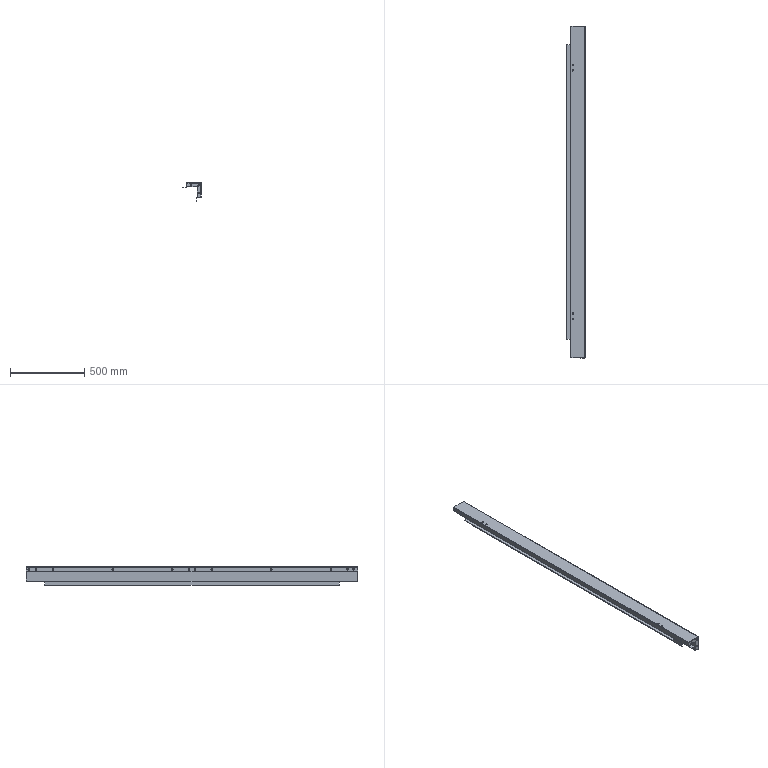Component | SolidWorks | 10RightFrontColumn-1 | 1 solid | 133 faces | volume 1330262 mm3 | cylinder 77 | plane 54 | spline 2 | commonest cylinder face diameters 10 x63 6 x7 2 x7